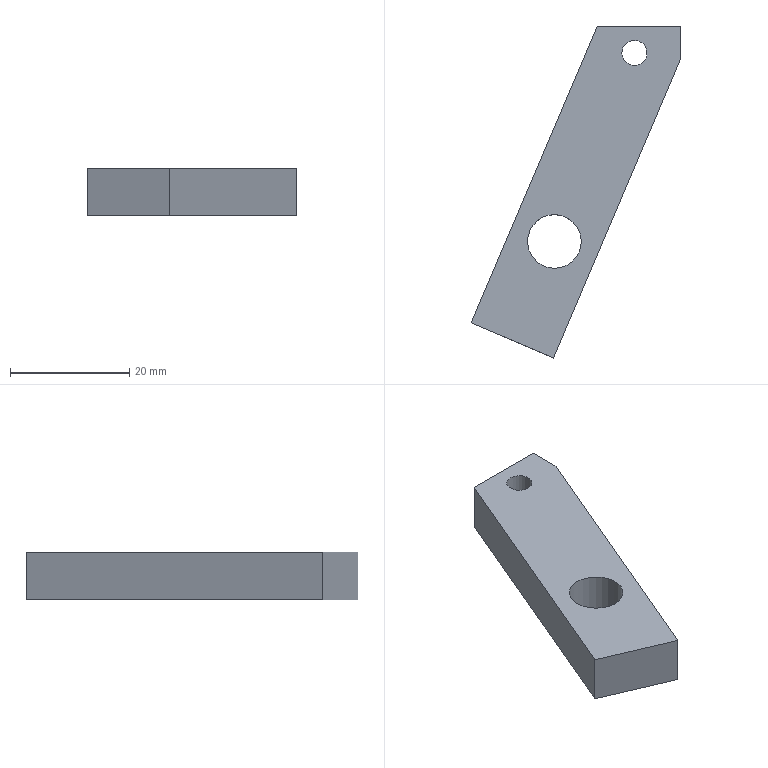Component | SolidWorks | PointedHeadDispensingCylinderConnector-2 | 1 solid | 11 faces | box 35.1 x 55.57 x 8 mm | volume 6193 mm3 | plane 7 | cylinder 4 | commonest cylinder face diameters 4.2 x2 9 x2
build123d program:
from build123d import *

# Parameters (mm, degrees)
SKETCH1_W          = 15
SKETCH1_H          = 52
EXTRUDE1_DEPTH     = 8
SKETCH2_R          = 4.5
CUT_EXTRUDE1_DEPTH = 55.708
CUT_EXTRUDE2_DEPTH = 55.708
SKETCH4_R          = 2.1
CUT_EXTRUDE3_DEPTH = 55.708
SKETCH5_W          = 15
SKETCH5_H          = 8
EXTRUDE2_DEPTH     = 10


with BuildPart() as part:
    # Sketch1 → Extrude1 (new body)
    with BuildSketch(Plane.XY):
        with Locations((7.5, -26)):
            Rectangle(SKETCH1_W, SKETCH1_H)
    extrude(amount=EXTRUDE1_DEPTH)

    # Sketch2 → Cut-Extrude1 (cut, through all)
    with BuildSketch(Plane.XY.offset(8)):
        with Locations((7.5, -44)):
            Circle(SKETCH2_R)
    extrude(amount=-CUT_EXTRUDE1_DEPTH, mode=Mode.SUBTRACT)

    # Sketch3 → Cut-Extrude2 (cut, through all)
    with BuildSketch(Plane(origin=(0, 0, 0), x_dir=(-1, 0, 0), z_dir=(0, 0, -1))):
        Polygon((-12.887, -2.53), (-15, -7.508), (-15, 0), (0, 0), (0, -8), align=None)
    extrude(amount=-CUT_EXTRUDE2_DEPTH, mode=Mode.SUBTRACT)

    # Sketch4 → Cut-Extrude3 (cut, through all)
    with BuildSketch(Plane(origin=(0, 0, 0), x_dir=(-1, 0, 0), z_dir=(0, 0, -1))):
        with Locations((-7.5, -9.705)):
            Circle(SKETCH4_R)
    extrude(amount=-CUT_EXTRUDE3_DEPTH, mode=Mode.SUBTRACT)

    # Sketch5 → Extrude2 (add)
    with BuildSketch(Plane.XZ.offset(52)):
        with Locations((7.5, 4)):
            Rectangle(SKETCH5_W, SKETCH5_H)
    extrude(amount=EXTRUDE2_DEPTH)


solid = part.part

# Placed as in the assembly
solid = solid.moved(Location((-1.195, 89.236, -85.887), (0, 0, -23)))
STEP:
#1=CARTESIAN_POINT('',(0.1516,3.014,-3.066));
#2=VERTEX_POINT('',#1);
#3=CARTESIAN_POINT('',(-0.0006379,3.078,-3.066));
#4=VERTEX_POINT('',#3);
#5=CARTESIAN_POINT('',(0.07547,3.046,-3.066));
#6=DIRECTION('',(0.,0.,-1.));
#7=DIRECTION('',(-0.9205,0.3907,0.));
#8=AXIS2_PLACEMENT_3D('',#5,#6,#7);
#9=CIRCLE('',#8,0.08268);
#10=EDGE_CURVE('',#2,#4,#9,.T.);
#11=ORIENTED_EDGE('',*,*,#10,.F.);
#12=CARTESIAN_POINT('',(0.1516,3.014,-3.381));
#13=VERTEX_POINT('',#12);
#14=CARTESIAN_POINT('',(0.1516,3.014,-3.066));
#15=DIRECTION('',(0.,0.,-1.));
#16=VECTOR('',#15,39.37);
#17=LINE('',#14,#16);
#18=EDGE_CURVE('',#2,#13,#17,.T.);
#19=ORIENTED_EDGE('',*,*,#18,.T.);
#20=CARTESIAN_POINT('',(-0.0006379,3.078,-3.381));
#21=VERTEX_POINT('',#20);
#22=CARTESIAN_POINT('',(0.07547,3.046,-3.381));
#23=DIRECTION('',(0.,0.,-1.));
#24=DIRECTION('',(-0.9205,0.3907,0.));
#25=AXIS2_PLACEMENT_3D('',#22,#23,#24);
#26=CIRCLE('',#25,0.08268);
#27=EDGE_CURVE('',#13,#21,#26,.T.);
#28=ORIENTED_EDGE('',*,*,#27,.T.);
#29=CARTESIAN_POINT('',(-0.0006379,3.078,-3.066));
#30=DIRECTION('',(0.,0.,-1.));
#31=VECTOR('',#30,39.37);
#32=LINE('',#29,#31);
#33=EDGE_CURVE('',#4,#21,#32,.T.);
#34=ORIENTED_EDGE('',*,*,#33,.F.);
#35=EDGE_LOOP('',(#11,#19,#28,#34));
#36=FACE_OUTER_BOUND('',#35,.T.);
#37=CARTESIAN_POINT('',(0.07547,3.046,-3.066));
#38=DIRECTION('',(0.,0.,-1.));
#39=DIRECTION('',(-0.9205,0.3907,0.));
#40=AXIS2_PLACEMENT_3D('',#37,#38,#39);
#41=CYLINDRICAL_SURFACE('',#40,0.08268);
#42=ADVANCED_FACE('',(#36),#41,.F.);
#43=CARTESIAN_POINT('',(-0.6152,1.873,-3.381));
#44=VERTEX_POINT('',#43);
#45=CARTESIAN_POINT('',(-0.289,1.734,-3.381));
#46=VERTEX_POINT('',#45);
#47=CARTESIAN_POINT('',(-0.4521,1.803,-3.381));
#48=DIRECTION('',(0.,0.,1.));
#49=DIRECTION('',(0.9205,-0.3907,0.));
#50=AXIS2_PLACEMENT_3D('',#47,#48,#49);
#51=CIRCLE('',#50,0.1772);
#52=EDGE_CURVE('',#44,#46,#51,.T.);
#53=ORIENTED_EDGE('',*,*,#52,.F.);
#54=CARTESIAN_POINT('',(-0.6152,1.873,-3.066));
#55=VERTEX_POINT('',#54);
#56=CARTESIAN_POINT('',(-0.6152,1.873,-3.381));
#57=DIRECTION('',(0.,0.,1.));
#58=VECTOR('',#57,39.37);
#59=LINE('',#56,#58);
#60=EDGE_CURVE('',#44,#55,#59,.T.);
#61=ORIENTED_EDGE('',*,*,#60,.T.);
#62=CARTESIAN_POINT('',(-0.289,1.734,-3.066));
#63=VERTEX_POINT('',#62);
#64=CARTESIAN_POINT('',(-0.4521,1.803,-3.066));
#65=DIRECTION('',(0.,0.,1.));
#66=DIRECTION('',(0.9205,-0.3907,0.));
#67=AXIS2_PLACEMENT_3D('',#64,#65,#66);
#68=CIRCLE('',#67,0.1772);
#69=EDGE_CURVE('',#55,#63,#68,.T.);
#70=ORIENTED_EDGE('',*,*,#69,.T.);
#71=CARTESIAN_POINT('',(-0.289,1.734,-3.381));
#72=DIRECTION('',(0.,0.,1.));
#73=VECTOR('',#72,39.37);
#74=LINE('',#71,#73);
#75=EDGE_CURVE('',#46,#63,#74,.T.);
#76=ORIENTED_EDGE('',*,*,#75,.F.);
#77=EDGE_LOOP('',(#53,#61,#70,#76));
#78=FACE_OUTER_BOUND('',#77,.T.);
#79=CARTESIAN_POINT('',(-0.4521,1.803,-3.381));
#80=DIRECTION('',(0.,0.,1.));
#81=DIRECTION('',(0.9205,-0.3907,0.));
#82=AXIS2_PLACEMENT_3D('',#79,#80,#81);
#83=CYLINDRICAL_SURFACE('',#82,0.1772);
#84=ADVANCED_FACE('',(#78),#83,.F.);
#85=CARTESIAN_POINT('',(-0.1701,3.223,-3.066));
#86=VERTEX_POINT('',#85);
#87=CARTESIAN_POINT('',(-1.001,1.266,-3.066));
#88=VERTEX_POINT('',#87);
#89=CARTESIAN_POINT('',(-0.04704,3.513,-3.066));
#90=DIRECTION('',(-0.3907,-0.9205,0.));
#91=VECTOR('',#90,39.37);
#92=LINE('',#89,#91);
#93=EDGE_CURVE('',#86,#88,#92,.T.);
#94=ORIENTED_EDGE('',*,*,#93,.F.);
#95=CARTESIAN_POINT('',(-0.1701,3.223,-3.381));
#96=VERTEX_POINT('',#95);
#97=CARTESIAN_POINT('',(-0.1701,3.223,-3.066));
#98=DIRECTION('',(0.,0.,-1.));
#99=VECTOR('',#98,39.37);
#100=LINE('',#97,#99);
#101=EDGE_CURVE('',#86,#96,#100,.T.);
#102=ORIENTED_EDGE('',*,*,#101,.T.);
#103=CARTESIAN_POINT('',(-1.001,1.266,-3.381));
#104=VERTEX_POINT('',#103);
#105=CARTESIAN_POINT('',(-0.04704,3.513,-3.381));
#106=DIRECTION('',(-0.3907,-0.9205,0.));
#107=VECTOR('',#106,39.37);
#108=LINE('',#105,#107);
#109=EDGE_CURVE('',#96,#104,#108,.T.);
#110=ORIENTED_EDGE('',*,*,#109,.T.);
#111=CARTESIAN_POINT('',(-1.001,1.266,-3.066));
#112=DIRECTION('',(0.,0.,-1.));
#113=VECTOR('',#112,39.37);
#114=LINE('',#111,#113);
#115=EDGE_CURVE('',#88,#104,#114,.T.);
#116=ORIENTED_EDGE('',*,*,#115,.F.);
#117=EDGE_LOOP('',(#94,#102,#110,#116));
#118=FACE_OUTER_BOUND('',#117,.T.);
#119=CARTESIAN_POINT('',(-0.04704,3.513,-3.066));
#120=DIRECTION('',(0.9205,-0.3907,0.));
#121=DIRECTION('',(0.3907,0.9205,0.));
#122=AXIS2_PLACEMENT_3D('',#119,#120,#121);
#123=PLANE('',#122);
#124=ADVANCED_FACE('',(#118),#123,.F.);
#125=CARTESIAN_POINT('',(-0.4572,1.036,-3.381));
#126=VERTEX_POINT('',#125);
#127=CARTESIAN_POINT('',(0.3811,3.01,-3.381));
#128=VERTEX_POINT('',#127);
#129=CARTESIAN_POINT('',(0.4966,3.282,-3.381));
#130=DIRECTION('',(0.3907,0.9205,0.));
#131=VECTOR('',#130,39.37);
#132=LINE('',#129,#131);
#133=EDGE_CURVE('',#126,#128,#132,.T.);
#134=ORIENTED_EDGE('',*,*,#133,.T.);
#135=CARTESIAN_POINT('',(0.3811,3.01,-3.066));
#136=VERTEX_POINT('',#135);
#137=CARTESIAN_POINT('',(0.3811,3.01,-3.066));
#138=DIRECTION('',(0.,0.,-1.));
#139=VECTOR('',#138,39.37);
#140=LINE('',#137,#139);
#141=EDGE_CURVE('',#136,#128,#140,.T.);
#142=ORIENTED_EDGE('',*,*,#141,.F.);
#143=CARTESIAN_POINT('',(-0.4572,1.036,-3.066));
#144=VERTEX_POINT('',#143);
#145=CARTESIAN_POINT('',(0.4966,3.282,-3.066));
#146=DIRECTION('',(0.3907,0.9205,0.));
#147=VECTOR('',#146,39.37);
#148=LINE('',#145,#147);
#149=EDGE_CURVE('',#144,#136,#148,.T.);
#150=ORIENTED_EDGE('',*,*,#149,.F.);
#151=CARTESIAN_POINT('',(-0.4572,1.036,-3.381));
#152=DIRECTION('',(0.,0.,1.));
#153=VECTOR('',#152,39.37);
#154=LINE('',#151,#153);
#155=EDGE_CURVE('',#126,#144,#154,.T.);
#156=ORIENTED_EDGE('',*,*,#155,.F.);
#157=EDGE_LOOP('',(#134,#142,#150,#156));
#158=FACE_OUTER_BOUND('',#157,.T.);
#159=CARTESIAN_POINT('',(0.4966,3.282,-3.066));
#160=DIRECTION('',(-0.9205,0.3907,0.));
#161=DIRECTION('',(-0.3907,-0.9205,0.));
#162=AXIS2_PLACEMENT_3D('',#159,#160,#161);
#163=PLANE('',#162);
#164=ADVANCED_FACE('',(#158),#163,.F.);
#165=CARTESIAN_POINT('',(0.07547,3.046,-3.066));
#166=DIRECTION('',(0.,0.,-1.));
#167=DIRECTION('',(-0.9205,0.3907,0.));
#168=AXIS2_PLACEMENT_3D('',#165,#166,#167);
#169=CIRCLE('',#168,0.08268);
#170=EDGE_CURVE('',#4,#2,#169,.T.);
#171=ORIENTED_EDGE('',*,*,#170,.T.);
#172=ORIENTED_EDGE('',*,*,#10,.T.);
#173=EDGE_LOOP('',(#171,#172));
#174=FACE_BOUND('',#173,.T.);
#175=CARTESIAN_POINT('',(0.3811,3.223,-3.066));
#176=VERTEX_POINT('',#175);
#177=CARTESIAN_POINT('',(-0.1701,3.223,-3.066));
#178=DIRECTION('',(-1.,0.,0.));
#179=VECTOR('',#178,39.37);
#180=LINE('',#177,#179);
#181=EDGE_CURVE('',#176,#86,#180,.T.);
#182=ORIENTED_EDGE('',*,*,#181,.T.);
#183=ORIENTED_EDGE('',*,*,#93,.T.);
#184=CARTESIAN_POINT('',(-0.4572,1.036,-3.066));
#185=DIRECTION('',(-0.9205,0.3907,0.));
#186=VECTOR('',#185,39.37);
#187=LINE('',#184,#186);
#188=EDGE_CURVE('',#144,#88,#187,.T.);
#189=ORIENTED_EDGE('',*,*,#188,.F.);
#190=ORIENTED_EDGE('',*,*,#149,.T.);
#191=CARTESIAN_POINT('',(0.3811,3.223,-3.066));
#192=DIRECTION('',(0.,1.,0.));
#193=VECTOR('',#192,39.37);
#194=LINE('',#191,#193);
#195=EDGE_CURVE('',#136,#176,#194,.T.);
#196=ORIENTED_EDGE('',*,*,#195,.T.);
#197=EDGE_LOOP('',(#182,#183,#189,#190,#196));
#198=FACE_OUTER_BOUND('',#197,.T.);
#199=CARTESIAN_POINT('',(-0.4521,1.803,-3.066));
#200=DIRECTION('',(0.,0.,1.));
#201=DIRECTION('',(0.9205,-0.3907,0.));
#202=AXIS2_PLACEMENT_3D('',#199,#200,#201);
#203=CIRCLE('',#202,0.1772);
#204=EDGE_CURVE('',#63,#55,#203,.T.);
#205=ORIENTED_EDGE('',*,*,#204,.F.);
#206=ORIENTED_EDGE('',*,*,#69,.F.);
#207=EDGE_LOOP('',(#205,#206));
#208=FACE_BOUND('',#207,.T.);
#209=CARTESIAN_POINT('',(-0.847,1.629,-3.066));
#210=DIRECTION('',(0.,0.,1.));
#211=DIRECTION('',(0.9205,-0.3907,0.));
#212=AXIS2_PLACEMENT_3D('',#209,#210,#211);
#213=PLANE('',#212);
#214=ADVANCED_FACE('',(#174,#198,#208),#213,.T.);
#215=CARTESIAN_POINT('',(0.07547,3.046,-3.381));
#216=DIRECTION('',(0.,0.,-1.));
#217=DIRECTION('',(-0.9205,0.3907,0.));
#218=AXIS2_PLACEMENT_3D('',#215,#216,#217);
#219=CIRCLE('',#218,0.08268);
#220=EDGE_CURVE('',#21,#13,#219,.T.);
#221=ORIENTED_EDGE('',*,*,#220,.F.);
#222=ORIENTED_EDGE('',*,*,#27,.F.);
#223=EDGE_LOOP('',(#221,#222));
#224=FACE_BOUND('',#223,.T.);
#225=CARTESIAN_POINT('',(-0.4521,1.803,-3.381));
#226=DIRECTION('',(0.,0.,1.));
#227=DIRECTION('',(0.9205,-0.3907,0.));
#228=AXIS2_PLACEMENT_3D('',#225,#226,#227);
#229=CIRCLE('',#228,0.1772);
#230=EDGE_CURVE('',#46,#44,#229,.T.);
#231=ORIENTED_EDGE('',*,*,#230,.T.);
#232=ORIENTED_EDGE('',*,*,#52,.T.);
#233=EDGE_LOOP('',(#231,#232));
#234=FACE_BOUND('',#233,.T.);
#235=ORIENTED_EDGE('',*,*,#109,.F.);
#236=CARTESIAN_POINT('',(0.3811,3.223,-3.381));
#237=VERTEX_POINT('',#236);
#238=CARTESIAN_POINT('',(-0.1701,3.223,-3.381));
#239=DIRECTION('',(-1.,0.,0.));
#240=VECTOR('',#239,39.37);
#241=LINE('',#238,#240);
#242=EDGE_CURVE('',#237,#96,#241,.T.);
#243=ORIENTED_EDGE('',*,*,#242,.F.);
#244=CARTESIAN_POINT('',(0.3811,3.223,-3.381));
#245=DIRECTION('',(0.,1.,0.));
#246=VECTOR('',#245,39.37);
#247=LINE('',#244,#246);
#248=EDGE_CURVE('',#128,#237,#247,.T.);
#249=ORIENTED_EDGE('',*,*,#248,.F.);
#250=ORIENTED_EDGE('',*,*,#133,.F.);
#251=CARTESIAN_POINT('',(-1.001,1.266,-3.381));
#252=DIRECTION('',(0.9205,-0.3907,0.));
#253=VECTOR('',#252,39.37);
#254=LINE('',#251,#253);
#255=EDGE_CURVE('',#104,#126,#254,.T.);
#256=ORIENTED_EDGE('',*,*,#255,.F.);
#257=EDGE_LOOP('',(#235,#243,#249,#250,#256));
#258=FACE_OUTER_BOUND('',#257,.T.);
#259=CARTESIAN_POINT('',(-0.847,1.629,-3.381));
#260=DIRECTION('',(0.,0.,1.));
#261=DIRECTION('',(0.9205,-0.3907,0.));
#262=AXIS2_PLACEMENT_3D('',#259,#260,#261);
#263=PLANE('',#262);
#264=ADVANCED_FACE('',(#224,#234,#258),#263,.F.);
#265=ORIENTED_EDGE('',*,*,#60,.F.);
#266=ORIENTED_EDGE('',*,*,#230,.F.);
#267=ORIENTED_EDGE('',*,*,#75,.T.);
#268=ORIENTED_EDGE('',*,*,#204,.T.);
#269=EDGE_LOOP('',(#265,#266,#267,#268));
#270=FACE_OUTER_BOUND('',#269,.T.);
#271=CARTESIAN_POINT('',(-0.4521,1.803,-3.381));
#272=DIRECTION('',(0.,0.,1.));
#273=DIRECTION('',(0.9205,-0.3907,0.));
#274=AXIS2_PLACEMENT_3D('',#271,#272,#273);
#275=CYLINDRICAL_SURFACE('',#274,0.1772);
#276=ADVANCED_FACE('',(#270),#275,.F.);
#277=ORIENTED_EDGE('',*,*,#242,.T.);
#278=ORIENTED_EDGE('',*,*,#101,.F.);
#279=ORIENTED_EDGE('',*,*,#181,.F.);
#280=CARTESIAN_POINT('',(0.3811,3.223,-3.066));
#281=DIRECTION('',(0.,0.,-1.));
#282=VECTOR('',#281,39.37);
#283=LINE('',#280,#282);
#284=EDGE_CURVE('',#176,#237,#283,.T.);
#285=ORIENTED_EDGE('',*,*,#284,.T.);
#286=EDGE_LOOP('',(#277,#278,#279,#285));
#287=FACE_OUTER_BOUND('',#286,.T.);
#288=CARTESIAN_POINT('',(-0.1701,3.223,-3.066));
#289=DIRECTION('',(0.,-1.,0.));
#290=DIRECTION('',(1.,0.,0.));
#291=AXIS2_PLACEMENT_3D('',#288,#289,#290);
#292=PLANE('',#291);
#293=ADVANCED_FACE('',(#287),#292,.F.);
#294=ORIENTED_EDGE('',*,*,#248,.T.);
#295=ORIENTED_EDGE('',*,*,#284,.F.);
#296=ORIENTED_EDGE('',*,*,#195,.F.);
#297=ORIENTED_EDGE('',*,*,#141,.T.);
#298=EDGE_LOOP('',(#294,#295,#296,#297));
#299=FACE_OUTER_BOUND('',#298,.T.);
#300=CARTESIAN_POINT('',(0.3811,3.223,-3.066));
#301=DIRECTION('',(-1.,0.,0.));
#302=DIRECTION('',(-0.,-1.,0.));
#303=AXIS2_PLACEMENT_3D('',#300,#301,#302);
#304=PLANE('',#303);
#305=ADVANCED_FACE('',(#299),#304,.F.);
#306=ORIENTED_EDGE('',*,*,#18,.F.);
#307=ORIENTED_EDGE('',*,*,#170,.F.);
#308=ORIENTED_EDGE('',*,*,#33,.T.);
#309=ORIENTED_EDGE('',*,*,#220,.T.);
#310=EDGE_LOOP('',(#306,#307,#308,#309));
#311=FACE_OUTER_BOUND('',#310,.T.);
#312=CARTESIAN_POINT('',(0.07547,3.046,-3.066));
#313=DIRECTION('',(0.,0.,-1.));
#314=DIRECTION('',(-0.9205,0.3907,0.));
#315=AXIS2_PLACEMENT_3D('',#312,#313,#314);
#316=CYLINDRICAL_SURFACE('',#315,0.08268);
#317=ADVANCED_FACE('',(#311),#316,.F.);
#318=ORIENTED_EDGE('',*,*,#115,.T.);
#319=ORIENTED_EDGE('',*,*,#255,.T.);
#320=ORIENTED_EDGE('',*,*,#155,.T.);
#321=ORIENTED_EDGE('',*,*,#188,.T.);
#322=EDGE_LOOP('',(#318,#319,#320,#321));
#323=FACE_OUTER_BOUND('',#322,.T.);
#324=CARTESIAN_POINT('',(-1.001,1.266,-3.381));
#325=DIRECTION('',(-0.3907,-0.9205,0.));
#326=DIRECTION('',(0.,0.,-1.));
#327=AXIS2_PLACEMENT_3D('',#324,#325,#326);
#328=PLANE('',#327);
#329=ADVANCED_FACE('',(#323),#328,.T.);
#330=CLOSED_SHELL('',(#42,#84,#124,#164,#214,#264,#276,#293,#305,#317,#329));
#331=MANIFOLD_SOLID_BREP('',#330);
#332=CARTESIAN_POINT('',(0.,0.,0.));
#333=DIRECTION('',(0.,0.,1.));
#334=DIRECTION('',(1.,0.,0.));
#335=AXIS2_PLACEMENT_3D('',#332,#333,#334);
#336=(LENGTH_UNIT()NAMED_UNIT(*)SI_UNIT($,.METRE.));
#337=LENGTH_MEASURE_WITH_UNIT(LENGTH_MEASURE(0.0254),#336);
#338=DIMENSIONAL_EXPONENTS(1.,0.,0.,0.,0.,0.,0.);
#339=(CONVERSION_BASED_UNIT('',#337)LENGTH_UNIT()NAMED_UNIT(#338));
#340=UNCERTAINTY_MEASURE_WITH_UNIT(LENGTH_MEASURE(0.00001),#339,'','');
#341=(NAMED_UNIT(*)PLANE_ANGLE_UNIT()SI_UNIT($,.RADIAN.));
#342=(NAMED_UNIT(*)SI_UNIT($,.STERADIAN.)SOLID_ANGLE_UNIT());
#343=(GEOMETRIC_REPRESENTATION_CONTEXT(3)GLOBAL_UNCERTAINTY_ASSIGNED_CONTEXT((#340))GLOBAL_UNIT_ASSIGNED_CONTEXT((#339,#341,#342))REPRESENTATION_CONTEXT('',''));
#344=ADVANCED_BREP_SHAPE_REPRESENTATION('',(#331,#335),#343);
#345=COLOUR_RGB('',0.7922,0.8196,0.9333);
#346=FILL_AREA_STYLE_COLOUR('',#345);
#347=FILL_AREA_STYLE('',(#346));
#348=SURFACE_STYLE_FILL_AREA(#347);
#349=SURFACE_SIDE_STYLE('',(#348));
#350=SURFACE_STYLE_USAGE(.BOTH.,#349);
#351=PRESENTATION_STYLE_ASSIGNMENT((#350));
#352=STYLED_ITEM('',(#351),#331);
#353=PRESENTATION_LAYER_ASSIGNMENT('','',(#352));
#354=(LENGTH_UNIT()NAMED_UNIT(*)SI_UNIT($,.METRE.));
#355=LENGTH_MEASURE_WITH_UNIT(LENGTH_MEASURE(0.0254),#354);
#356=DIMENSIONAL_EXPONENTS(1.,0.,0.,0.,0.,0.,0.);
#357=(CONVERSION_BASED_UNIT('',#355)LENGTH_UNIT()NAMED_UNIT(#356));
#358=UNCERTAINTY_MEASURE_WITH_UNIT(LENGTH_MEASURE(0.00001),#357,'','');
#359=(NAMED_UNIT(*)PLANE_ANGLE_UNIT()SI_UNIT($,.RADIAN.));
#360=(NAMED_UNIT(*)SI_UNIT($,.STERADIAN.)SOLID_ANGLE_UNIT());
#361=(GEOMETRIC_REPRESENTATION_CONTEXT(3)GLOBAL_UNCERTAINTY_ASSIGNED_CONTEXT((#358))GLOBAL_UNIT_ASSIGNED_CONTEXT((#357,#359,#360))REPRESENTATION_CONTEXT('',''));
#362=MECHANICAL_DESIGN_GEOMETRIC_PRESENTATION_REPRESENTATION('',(#352),#361);